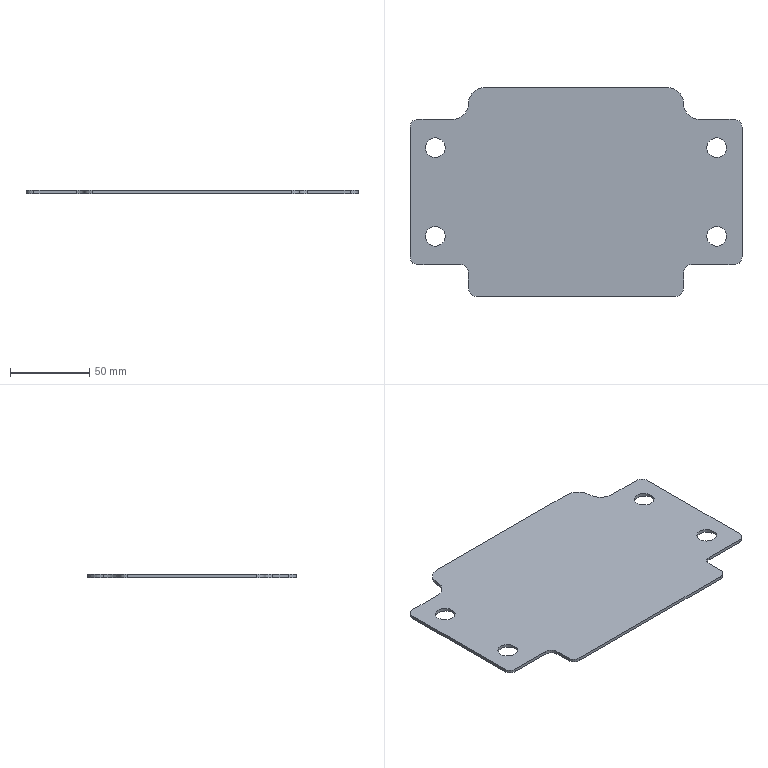CAM job | Mastercam | mm | 3 operations | part box 420 x 297 x 2
1. Contour (Ramp) | 2 - 2 平铣刀
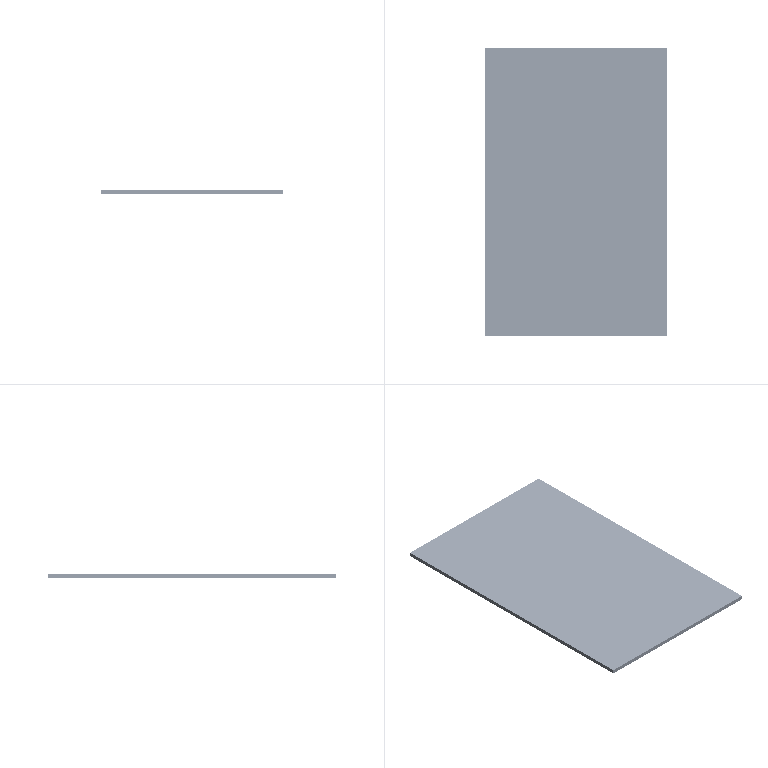2. Contour (2D chamfer) | 5 - 4 倒角刀
3. Contour (2D) | 2 - 2 平铣刀